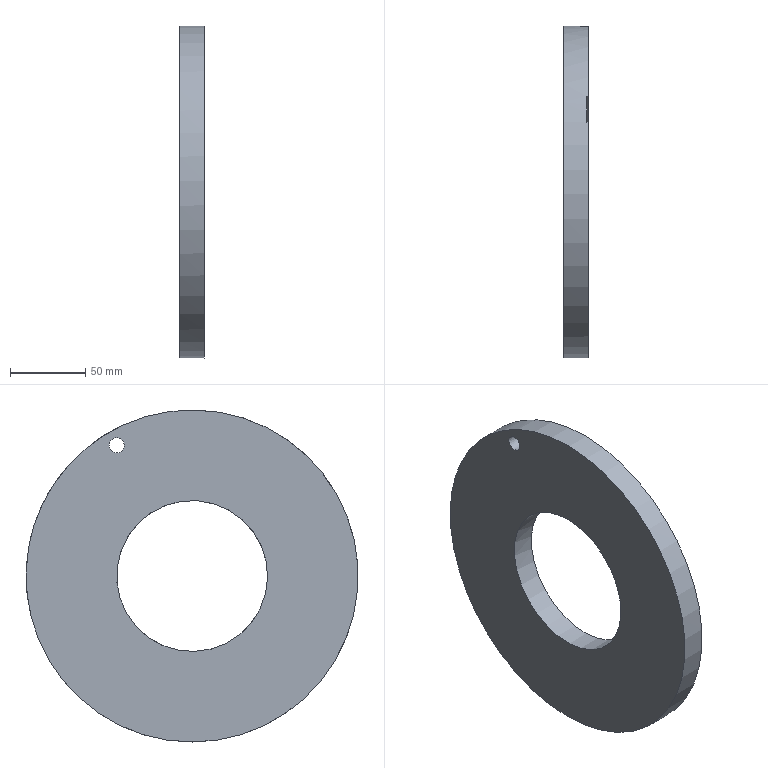Component | NX | SIM15_C4_AXIS | 1 solid | 8 faces | volume 480167 mm3 | plane 5 | cylinder 3 | commonest cylinder face diameters 220 x1 100 x1 10 x1